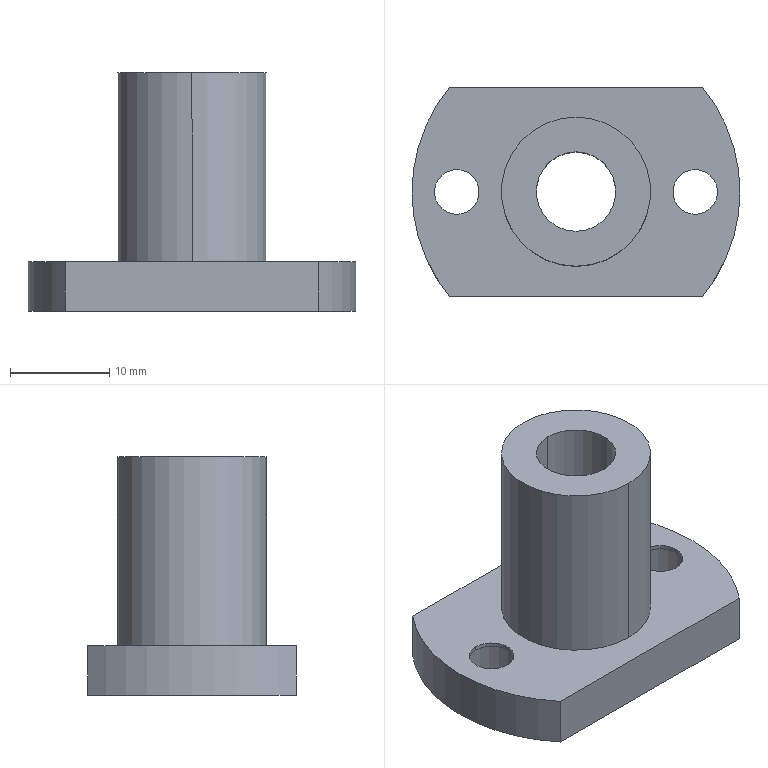Component | SolidWorks | LinearBearing8uu-1 | 1 solid | 21 faces | box 33 x 21 x 24 mm | volume 4890 mm3 | cylinder 14 | plane 7 | commonest cylinder face diameters 8 x6 4.5 x4 15 x2 33 x2
build123d program:
from build123d import *

# Parameters (mm, degrees)
SKETCH2_W                                         = 10.005
SKETCH2_H                                         = 30.735
SKETCH2_W_2                                       = 17.846
SKETCH2_H_2                                       = 33.574
CUT_EXTRUDE1_DEPTH                                = 10
HOLE_SIZE_ACCORDING_TO_HEXAGON_SOCKET_D           = 4.5
HOLE_SIZE_ACCORDING_TO_HEXAGON_SOCKET_DEPTH       = 22.25
HOLE_SIZE_ACCORDING_TO_HEXAGON_SOCKET_CBORE_D     = 8
HOLE_SIZE_ACCORDING_TO_HEXAGON_SOCKET_CBORE_DEPTH = 4.6
HOLE_SIZE_ACCORDING_TO_HEXAGON_SOCKET_TIP         = 1.352


with BuildPart() as part:
    # Sketch1 → Revolve1 (revolve)
    with BuildSketch(Plane.XY, mode=Mode.PRIVATE) as revolve1_sk:
        Polygon((0, 4), (0, 16.5), (5, 16.5), (5, 7.5), (24, 7.5), (24, 4), align=None)
    revolve(revolve1_sk.sketch.rotate(Axis((-24.161, 0, 0), (1, 0, 0)), 90), axis=Axis((-24.161, 0, 0), (1, 0, 0)))

    # Sketch2 → Cut-Extrude1 (cut)
    with BuildSketch(Plane.ZY):
        with Locations((-15.502, 0.676)):
            Rectangle(SKETCH2_W, SKETCH2_H)
        with Locations((19.423, 0.9239)):
            Rectangle(SKETCH2_W_2, SKETCH2_H_2)
    extrude(amount=-CUT_EXTRUDE1_DEPTH, mode=Mode.SUBTRACT)

    # Hole Size _According to_ Hexagon Socket
    with Locations(Plane(origin=(0, 12, 0), x_dir=(0, 0, -1), z_dir=(-1, 0, 0))):
        with Locations((0, 0), (0, 24)):
            CounterBoreHole(HOLE_SIZE_ACCORDING_TO_HEXAGON_SOCKET_D / 2, HOLE_SIZE_ACCORDING_TO_HEXAGON_SOCKET_CBORE_D / 2, HOLE_SIZE_ACCORDING_TO_HEXAGON_SOCKET_CBORE_DEPTH, depth=HOLE_SIZE_ACCORDING_TO_HEXAGON_SOCKET_DEPTH)
            with Locations((0, 0, -(HOLE_SIZE_ACCORDING_TO_HEXAGON_SOCKET_DEPTH + HOLE_SIZE_ACCORDING_TO_HEXAGON_SOCKET_TIP / 2))):  # 118° drill point
                Cone(0, HOLE_SIZE_ACCORDING_TO_HEXAGON_SOCKET_D / 2, HOLE_SIZE_ACCORDING_TO_HEXAGON_SOCKET_TIP, mode=Mode.SUBTRACT)


solid = part.part

# Placed as in the assembly
solid = solid.moved(Location((30, -219.228, 51), (90, 0, 90)))
STEP:
#1=COLOUR_RGB('',0.7922,0.8196,0.9333);
#2=FILL_AREA_STYLE_COLOUR('',#1);
#3=FILL_AREA_STYLE('',(#2));
#4=SURFACE_STYLE_FILL_AREA(#3);
#5=SURFACE_SIDE_STYLE('',(#4));
#6=SURFACE_STYLE_USAGE(.BOTH.,#5);
#7=PRESENTATION_STYLE_ASSIGNMENT((#6));
#8=CARTESIAN_POINT('',(0.7087,-8.474,2.189));
#9=VERTEX_POINT('',#8);
#10=CARTESIAN_POINT('',(0.7087,-8.789,2.189));
#11=VERTEX_POINT('',#10);
#12=CARTESIAN_POINT('',(0.7087,-8.631,2.189));
#13=DIRECTION('',(0.,0.,-1.));
#14=DIRECTION('',(0.,-1.,0.));
#15=AXIS2_PLACEMENT_3D('',#12,#13,#14);
#16=CIRCLE('',#15,0.1575);
#17=EDGE_CURVE('',#9,#11,#16,.T.);
#18=ORIENTED_EDGE('',*,*,#17,.F.);
#19=CARTESIAN_POINT('',(0.7087,-8.474,2.008));
#20=VERTEX_POINT('',#19);
#21=CARTESIAN_POINT('',(0.7087,-8.474,2.008));
#22=DIRECTION('',(0.,0.,-1.));
#23=VECTOR('',#22,39.37);
#24=LINE('',#21,#23);
#25=EDGE_CURVE('',#9,#20,#24,.T.);
#26=ORIENTED_EDGE('',*,*,#25,.T.);
#27=CARTESIAN_POINT('',(0.7087,-8.789,2.008));
#28=VERTEX_POINT('',#27);
#29=CARTESIAN_POINT('',(0.7087,-8.631,2.008));
#30=DIRECTION('',(0.,0.,-1.));
#31=DIRECTION('',(0.,-1.,0.));
#32=AXIS2_PLACEMENT_3D('',#29,#30,#31);
#33=CIRCLE('',#32,0.1575);
#34=EDGE_CURVE('',#20,#28,#33,.T.);
#35=ORIENTED_EDGE('',*,*,#34,.T.);
#36=CARTESIAN_POINT('',(0.7087,-8.789,2.008));
#37=DIRECTION('',(0.,0.,-1.));
#38=VECTOR('',#37,39.37);
#39=LINE('',#36,#38);
#40=EDGE_CURVE('',#11,#28,#39,.T.);
#41=ORIENTED_EDGE('',*,*,#40,.F.);
#42=EDGE_LOOP('',(#18,#26,#35,#41));
#43=FACE_OUTER_BOUND('',#42,.T.);
#44=CARTESIAN_POINT('',(0.7087,-8.631,2.008));
#45=DIRECTION('',(0.,0.,-1.));
#46=DIRECTION('',(0.,-1.,0.));
#47=AXIS2_PLACEMENT_3D('',#44,#45,#46);
#48=CYLINDRICAL_SURFACE('',#47,0.1575);
#49=ADVANCED_FACE('',(#43),#48,.F.);
#50=CARTESIAN_POINT('',(0.7087,-8.542,2.205));
#51=VERTEX_POINT('',#50);
#52=CARTESIAN_POINT('',(0.7087,-8.72,2.205));
#53=VERTEX_POINT('',#52);
#54=CARTESIAN_POINT('',(0.7087,-8.631,2.205));
#55=DIRECTION('',(0.,0.,-1.));
#56=DIRECTION('',(0.,-1.,0.));
#57=AXIS2_PLACEMENT_3D('',#54,#55,#56);
#58=CIRCLE('',#57,0.08858);
#59=EDGE_CURVE('',#51,#53,#58,.T.);
#60=ORIENTED_EDGE('',*,*,#59,.F.);
#61=CARTESIAN_POINT('',(0.7087,-8.542,2.189));
#62=VERTEX_POINT('',#61);
#63=CARTESIAN_POINT('',(0.7087,-8.542,2.008));
#64=DIRECTION('',(0.,0.,-1.));
#65=VECTOR('',#64,39.37);
#66=LINE('',#63,#65);
#67=EDGE_CURVE('',#51,#62,#66,.T.);
#68=ORIENTED_EDGE('',*,*,#67,.T.);
#69=CARTESIAN_POINT('',(0.7087,-8.72,2.189));
#70=VERTEX_POINT('',#69);
#71=CARTESIAN_POINT('',(0.7087,-8.631,2.189));
#72=DIRECTION('',(0.,0.,-1.));
#73=DIRECTION('',(0.,-1.,0.));
#74=AXIS2_PLACEMENT_3D('',#71,#72,#73);
#75=CIRCLE('',#74,0.08858);
#76=EDGE_CURVE('',#62,#70,#75,.T.);
#77=ORIENTED_EDGE('',*,*,#76,.T.);
#78=CARTESIAN_POINT('',(0.7087,-8.72,2.008));
#79=DIRECTION('',(0.,0.,-1.));
#80=VECTOR('',#79,39.37);
#81=LINE('',#78,#80);
#82=EDGE_CURVE('',#53,#70,#81,.T.);
#83=ORIENTED_EDGE('',*,*,#82,.F.);
#84=EDGE_LOOP('',(#60,#68,#77,#83));
#85=FACE_OUTER_BOUND('',#84,.T.);
#86=CARTESIAN_POINT('',(0.7087,-8.631,2.008));
#87=DIRECTION('',(0.,0.,-1.));
#88=DIRECTION('',(0.,-1.,0.));
#89=AXIS2_PLACEMENT_3D('',#86,#87,#88);
#90=CYLINDRICAL_SURFACE('',#89,0.08858);
#91=ADVANCED_FACE('',(#85),#90,.F.);
#92=CARTESIAN_POINT('',(1.654,-8.474,2.189));
#93=VERTEX_POINT('',#92);
#94=CARTESIAN_POINT('',(1.654,-8.789,2.189));
#95=VERTEX_POINT('',#94);
#96=CARTESIAN_POINT('',(1.654,-8.631,2.189));
#97=DIRECTION('',(0.,0.,-1.));
#98=DIRECTION('',(0.,-1.,0.));
#99=AXIS2_PLACEMENT_3D('',#96,#97,#98);
#100=CIRCLE('',#99,0.1575);
#101=EDGE_CURVE('',#93,#95,#100,.T.);
#102=ORIENTED_EDGE('',*,*,#101,.F.);
#103=CARTESIAN_POINT('',(1.654,-8.474,2.008));
#104=VERTEX_POINT('',#103);
#105=CARTESIAN_POINT('',(1.654,-8.474,2.008));
#106=DIRECTION('',(0.,0.,-1.));
#107=VECTOR('',#106,39.37);
#108=LINE('',#105,#107);
#109=EDGE_CURVE('',#93,#104,#108,.T.);
#110=ORIENTED_EDGE('',*,*,#109,.T.);
#111=CARTESIAN_POINT('',(1.654,-8.789,2.008));
#112=VERTEX_POINT('',#111);
#113=CARTESIAN_POINT('',(1.654,-8.631,2.008));
#114=DIRECTION('',(0.,0.,-1.));
#115=DIRECTION('',(0.,-1.,0.));
#116=AXIS2_PLACEMENT_3D('',#113,#114,#115);
#117=CIRCLE('',#116,0.1575);
#118=EDGE_CURVE('',#104,#112,#117,.T.);
#119=ORIENTED_EDGE('',*,*,#118,.T.);
#120=CARTESIAN_POINT('',(1.654,-8.789,2.008));
#121=DIRECTION('',(0.,0.,-1.));
#122=VECTOR('',#121,39.37);
#123=LINE('',#120,#122);
#124=EDGE_CURVE('',#95,#112,#123,.T.);
#125=ORIENTED_EDGE('',*,*,#124,.F.);
#126=EDGE_LOOP('',(#102,#110,#119,#125));
#127=FACE_OUTER_BOUND('',#126,.T.);
#128=CARTESIAN_POINT('',(1.654,-8.631,2.008));
#129=DIRECTION('',(0.,0.,-1.));
#130=DIRECTION('',(0.,-1.,0.));
#131=AXIS2_PLACEMENT_3D('',#128,#129,#130);
#132=CYLINDRICAL_SURFACE('',#131,0.1575);
#133=ADVANCED_FACE('',(#127),#132,.F.);
#134=CARTESIAN_POINT('',(1.654,-8.542,2.205));
#135=VERTEX_POINT('',#134);
#136=CARTESIAN_POINT('',(1.654,-8.72,2.205));
#137=VERTEX_POINT('',#136);
#138=CARTESIAN_POINT('',(1.654,-8.631,2.205));
#139=DIRECTION('',(0.,0.,-1.));
#140=DIRECTION('',(0.,-1.,0.));
#141=AXIS2_PLACEMENT_3D('',#138,#139,#140);
#142=CIRCLE('',#141,0.08858);
#143=EDGE_CURVE('',#135,#137,#142,.T.);
#144=ORIENTED_EDGE('',*,*,#143,.F.);
#145=CARTESIAN_POINT('',(1.654,-8.542,2.189));
#146=VERTEX_POINT('',#145);
#147=CARTESIAN_POINT('',(1.654,-8.542,2.008));
#148=DIRECTION('',(0.,0.,-1.));
#149=VECTOR('',#148,39.37);
#150=LINE('',#147,#149);
#151=EDGE_CURVE('',#135,#146,#150,.T.);
#152=ORIENTED_EDGE('',*,*,#151,.T.);
#153=CARTESIAN_POINT('',(1.654,-8.72,2.189));
#154=VERTEX_POINT('',#153);
#155=CARTESIAN_POINT('',(1.654,-8.631,2.189));
#156=DIRECTION('',(0.,0.,-1.));
#157=DIRECTION('',(0.,-1.,0.));
#158=AXIS2_PLACEMENT_3D('',#155,#156,#157);
#159=CIRCLE('',#158,0.08858);
#160=EDGE_CURVE('',#146,#154,#159,.T.);
#161=ORIENTED_EDGE('',*,*,#160,.T.);
#162=CARTESIAN_POINT('',(1.654,-8.72,2.008));
#163=DIRECTION('',(0.,0.,-1.));
#164=VECTOR('',#163,39.37);
#165=LINE('',#162,#164);
#166=EDGE_CURVE('',#137,#154,#165,.T.);
#167=ORIENTED_EDGE('',*,*,#166,.F.);
#168=EDGE_LOOP('',(#144,#152,#161,#167));
#169=FACE_OUTER_BOUND('',#168,.T.);
#170=CARTESIAN_POINT('',(1.654,-8.631,2.008));
#171=DIRECTION('',(0.,0.,-1.));
#172=DIRECTION('',(0.,-1.,0.));
#173=AXIS2_PLACEMENT_3D('',#170,#171,#172);
#174=CYLINDRICAL_SURFACE('',#173,0.08858);
#175=ADVANCED_FACE('',(#169),#174,.F.);
#176=CARTESIAN_POINT('',(1.181,-8.926,2.953));
#177=VERTEX_POINT('',#176);
#178=CARTESIAN_POINT('',(1.181,-8.336,2.953));
#179=VERTEX_POINT('',#178);
#180=CARTESIAN_POINT('',(1.181,-8.631,2.953));
#181=DIRECTION('',(0.,0.,-1.));
#182=DIRECTION('',(-0.,-1.,0.));
#183=AXIS2_PLACEMENT_3D('',#180,#181,#182);
#184=CIRCLE('',#183,0.2953);
#185=EDGE_CURVE('',#177,#179,#184,.T.);
#186=ORIENTED_EDGE('',*,*,#185,.T.);
#187=CARTESIAN_POINT('',(1.181,-8.336,2.205));
#188=VERTEX_POINT('',#187);
#189=CARTESIAN_POINT('',(1.181,-8.336,1.057));
#190=DIRECTION('',(0.,0.,-1.));
#191=VECTOR('',#190,39.37);
#192=LINE('',#189,#191);
#193=EDGE_CURVE('',#179,#188,#192,.T.);
#194=ORIENTED_EDGE('',*,*,#193,.T.);
#195=CARTESIAN_POINT('',(1.181,-8.926,2.205));
#196=VERTEX_POINT('',#195);
#197=CARTESIAN_POINT('',(1.181,-8.631,2.205));
#198=DIRECTION('',(0.,0.,-1.));
#199=DIRECTION('',(-0.,-1.,0.));
#200=AXIS2_PLACEMENT_3D('',#197,#198,#199);
#201=CIRCLE('',#200,0.2953);
#202=EDGE_CURVE('',#196,#188,#201,.T.);
#203=ORIENTED_EDGE('',*,*,#202,.F.);
#204=CARTESIAN_POINT('',(1.181,-8.926,1.057));
#205=DIRECTION('',(0.,0.,-1.));
#206=VECTOR('',#205,39.37);
#207=LINE('',#204,#206);
#208=EDGE_CURVE('',#177,#196,#207,.T.);
#209=ORIENTED_EDGE('',*,*,#208,.F.);
#210=EDGE_LOOP('',(#186,#194,#203,#209));
#211=FACE_OUTER_BOUND('',#210,.T.);
#212=CARTESIAN_POINT('',(1.181,-8.631,1.057));
#213=DIRECTION('',(0.,0.,-1.));
#214=DIRECTION('',(-0.,-1.,-0.));
#215=AXIS2_PLACEMENT_3D('',#212,#213,#214);
#216=CYLINDRICAL_SURFACE('',#215,0.2953);
#217=ADVANCED_FACE('',(#211),#216,.T.);
#218=CARTESIAN_POINT('',(1.181,-8.474,2.953));
#219=VERTEX_POINT('',#218);
#220=CARTESIAN_POINT('',(1.181,-8.789,2.953));
#221=VERTEX_POINT('',#220);
#222=CARTESIAN_POINT('',(1.181,-8.631,2.953));
#223=DIRECTION('',(0.,0.,-1.));
#224=DIRECTION('',(0.,-1.,0.));
#225=AXIS2_PLACEMENT_3D('',#222,#223,#224);
#226=CIRCLE('',#225,0.1575);
#227=EDGE_CURVE('',#219,#221,#226,.T.);
#228=ORIENTED_EDGE('',*,*,#227,.F.);
#229=CARTESIAN_POINT('',(1.181,-8.474,2.008));
#230=VERTEX_POINT('',#229);
#231=CARTESIAN_POINT('',(1.181,-8.474,1.057));
#232=DIRECTION('',(0.,0.,-1.));
#233=VECTOR('',#232,39.37);
#234=LINE('',#231,#233);
#235=EDGE_CURVE('',#219,#230,#234,.T.);
#236=ORIENTED_EDGE('',*,*,#235,.T.);
#237=CARTESIAN_POINT('',(1.181,-8.789,2.008));
#238=VERTEX_POINT('',#237);
#239=CARTESIAN_POINT('',(1.181,-8.631,2.008));
#240=DIRECTION('',(0.,0.,-1.));
#241=DIRECTION('',(0.,-1.,0.));
#242=AXIS2_PLACEMENT_3D('',#239,#240,#241);
#243=CIRCLE('',#242,0.1575);
#244=EDGE_CURVE('',#230,#238,#243,.T.);
#245=ORIENTED_EDGE('',*,*,#244,.T.);
#246=CARTESIAN_POINT('',(1.181,-8.789,1.057));
#247=DIRECTION('',(0.,0.,-1.));
#248=VECTOR('',#247,39.37);
#249=LINE('',#246,#248);
#250=EDGE_CURVE('',#221,#238,#249,.T.);
#251=ORIENTED_EDGE('',*,*,#250,.F.);
#252=EDGE_LOOP('',(#228,#236,#245,#251));
#253=FACE_OUTER_BOUND('',#252,.T.);
#254=CARTESIAN_POINT('',(1.181,-8.631,1.057));
#255=DIRECTION('',(0.,0.,-1.));
#256=DIRECTION('',(0.,-1.,0.));
#257=AXIS2_PLACEMENT_3D('',#254,#255,#256);
#258=CYLINDRICAL_SURFACE('',#257,0.1575);
#259=ADVANCED_FACE('',(#253),#258,.F.);
#260=CARTESIAN_POINT('',(1.682,-8.218,2.205));
#261=VERTEX_POINT('',#260);
#262=CARTESIAN_POINT('',(1.682,-9.044,2.205));
#263=VERTEX_POINT('',#262);
#264=CARTESIAN_POINT('',(1.181,-8.631,2.205));
#265=DIRECTION('',(0.,0.,-1.));
#266=DIRECTION('',(-0.,-1.,-0.));
#267=AXIS2_PLACEMENT_3D('',#264,#265,#266);
#268=CIRCLE('',#267,0.6496);
#269=EDGE_CURVE('',#261,#263,#268,.T.);
#270=ORIENTED_EDGE('',*,*,#269,.T.);
#271=CARTESIAN_POINT('',(1.682,-9.044,2.008));
#272=VERTEX_POINT('',#271);
#273=CARTESIAN_POINT('',(1.682,-9.044,1.057));
#274=DIRECTION('',(0.,0.,-1.));
#275=VECTOR('',#274,39.37);
#276=LINE('',#273,#275);
#277=EDGE_CURVE('',#263,#272,#276,.T.);
#278=ORIENTED_EDGE('',*,*,#277,.T.);
#279=CARTESIAN_POINT('',(1.682,-8.218,2.008));
#280=VERTEX_POINT('',#279);
#281=CARTESIAN_POINT('',(1.181,-8.631,2.008));
#282=DIRECTION('',(0.,0.,-1.));
#283=DIRECTION('',(-0.,-1.,-0.));
#284=AXIS2_PLACEMENT_3D('',#281,#282,#283);
#285=CIRCLE('',#284,0.6496);
#286=EDGE_CURVE('',#280,#272,#285,.T.);
#287=ORIENTED_EDGE('',*,*,#286,.F.);
#288=CARTESIAN_POINT('',(1.682,-8.218,1.057));
#289=DIRECTION('',(-0.,-0.,1.));
#290=VECTOR('',#289,39.37);
#291=LINE('',#288,#290);
#292=EDGE_CURVE('',#280,#261,#291,.T.);
#293=ORIENTED_EDGE('',*,*,#292,.T.);
#294=EDGE_LOOP('',(#270,#278,#287,#293));
#295=FACE_OUTER_BOUND('',#294,.T.);
#296=CARTESIAN_POINT('',(1.181,-8.631,1.057));
#297=DIRECTION('',(0.,0.,-1.));
#298=DIRECTION('',(-0.,-1.,-0.));
#299=AXIS2_PLACEMENT_3D('',#296,#297,#298);
#300=CYLINDRICAL_SURFACE('',#299,0.6496);
#301=ADVANCED_FACE('',(#295),#300,.T.);
#302=ORIENTED_EDGE('',*,*,#235,.F.);
#303=CARTESIAN_POINT('',(1.181,-8.631,2.953));
#304=DIRECTION('',(0.,0.,-1.));
#305=DIRECTION('',(0.,-1.,0.));
#306=AXIS2_PLACEMENT_3D('',#303,#304,#305);
#307=CIRCLE('',#306,0.1575);
#308=EDGE_CURVE('',#221,#219,#307,.T.);
#309=ORIENTED_EDGE('',*,*,#308,.F.);
#310=ORIENTED_EDGE('',*,*,#250,.T.);
#311=CARTESIAN_POINT('',(1.181,-8.631,2.008));
#312=DIRECTION('',(0.,0.,-1.));
#313=DIRECTION('',(0.,-1.,0.));
#314=AXIS2_PLACEMENT_3D('',#311,#312,#313);
#315=CIRCLE('',#314,0.1575);
#316=EDGE_CURVE('',#238,#230,#315,.T.);
#317=ORIENTED_EDGE('',*,*,#316,.T.);
#318=EDGE_LOOP('',(#302,#309,#310,#317));
#319=FACE_OUTER_BOUND('',#318,.T.);
#320=CARTESIAN_POINT('',(1.181,-8.631,1.057));
#321=DIRECTION('',(0.,0.,-1.));
#322=DIRECTION('',(0.,-1.,0.));
#323=AXIS2_PLACEMENT_3D('',#320,#321,#322);
#324=CYLINDRICAL_SURFACE('',#323,0.1575);
#325=ADVANCED_FACE('',(#319),#324,.F.);
#326=CARTESIAN_POINT('',(0.7087,-8.631,2.008));
#327=DIRECTION('',(0.,0.,-1.));
#328=DIRECTION('',(0.,-1.,0.));
#329=AXIS2_PLACEMENT_3D('',#326,#327,#328);
#330=CIRCLE('',#329,0.1575);
#331=EDGE_CURVE('',#28,#20,#330,.T.);
#332=ORIENTED_EDGE('',*,*,#331,.F.);
#333=ORIENTED_EDGE('',*,*,#34,.F.);
#334=EDGE_LOOP('',(#332,#333));
#335=FACE_BOUND('',#334,.T.);
#336=CARTESIAN_POINT('',(1.654,-8.631,2.008));
#337=DIRECTION('',(0.,0.,-1.));
#338=DIRECTION('',(0.,-1.,0.));
#339=AXIS2_PLACEMENT_3D('',#336,#337,#338);
#340=CIRCLE('',#339,0.1575);
#341=EDGE_CURVE('',#112,#104,#340,.T.);
#342=ORIENTED_EDGE('',*,*,#341,.F.);
#343=ORIENTED_EDGE('',*,*,#118,.F.);
#344=EDGE_LOOP('',(#342,#343));
#345=FACE_BOUND('',#344,.T.);
#346=ORIENTED_EDGE('',*,*,#316,.F.);
#347=ORIENTED_EDGE('',*,*,#244,.F.);
#348=EDGE_LOOP('',(#346,#347));
#349=FACE_BOUND('',#348,.T.);
#350=ORIENTED_EDGE('',*,*,#286,.T.);
#351=CARTESIAN_POINT('',(0.68,-9.044,2.008));
#352=VERTEX_POINT('',#351);
#353=CARTESIAN_POINT('',(0.4838,-9.044,2.008));
#354=DIRECTION('',(1.,-0.,0.));
#355=VECTOR('',#354,39.37);
#356=LINE('',#353,#355);
#357=EDGE_CURVE('',#352,#272,#356,.T.);
#358=ORIENTED_EDGE('',*,*,#357,.F.);
#359=CARTESIAN_POINT('',(0.68,-8.218,2.008));
#360=VERTEX_POINT('',#359);
#361=CARTESIAN_POINT('',(1.181,-8.631,2.008));
#362=DIRECTION('',(0.,0.,-1.));
#363=DIRECTION('',(-0.,-1.,-0.));
#364=AXIS2_PLACEMENT_3D('',#361,#362,#363);
#365=CIRCLE('',#364,0.6496);
#366=EDGE_CURVE('',#352,#360,#365,.T.);
#367=ORIENTED_EDGE('',*,*,#366,.T.);
#368=CARTESIAN_POINT('',(0.5495,-8.218,2.008));
#369=DIRECTION('',(-1.,0.,-0.));
#370=VECTOR('',#369,39.37);
#371=LINE('',#368,#370);
#372=EDGE_CURVE('',#280,#360,#371,.T.);
#373=ORIENTED_EDGE('',*,*,#372,.F.);
#374=EDGE_LOOP('',(#350,#358,#367,#373));
#375=FACE_OUTER_BOUND('',#374,.T.);
#376=CARTESIAN_POINT('',(1.024,-8.631,2.008));
#377=DIRECTION('',(-0.,-0.,1.));
#378=DIRECTION('',(0.,1.,0.));
#379=AXIS2_PLACEMENT_3D('',#376,#377,#378);
#380=PLANE('',#379);
#381=ADVANCED_FACE('',(#335,#345,#349,#375),#380,.F.);
#382=ORIENTED_EDGE('',*,*,#366,.F.);
#383=CARTESIAN_POINT('',(0.68,-9.044,2.205));
#384=VERTEX_POINT('',#383);
#385=CARTESIAN_POINT('',(0.68,-9.044,1.057));
#386=DIRECTION('',(-0.,-0.,1.));
#387=VECTOR('',#386,39.37);
#388=LINE('',#385,#387);
#389=EDGE_CURVE('',#352,#384,#388,.T.);
#390=ORIENTED_EDGE('',*,*,#389,.T.);
#391=CARTESIAN_POINT('',(0.68,-8.218,2.205));
#392=VERTEX_POINT('',#391);
#393=CARTESIAN_POINT('',(1.181,-8.631,2.205));
#394=DIRECTION('',(0.,0.,-1.));
#395=DIRECTION('',(-0.,-1.,-0.));
#396=AXIS2_PLACEMENT_3D('',#393,#394,#395);
#397=CIRCLE('',#396,0.6496);
#398=EDGE_CURVE('',#384,#392,#397,.T.);
#399=ORIENTED_EDGE('',*,*,#398,.T.);
#400=CARTESIAN_POINT('',(0.68,-8.218,1.057));
#401=DIRECTION('',(0.,0.,-1.));
#402=VECTOR('',#401,39.37);
#403=LINE('',#400,#402);
#404=EDGE_CURVE('',#392,#360,#403,.T.);
#405=ORIENTED_EDGE('',*,*,#404,.T.);
#406=EDGE_LOOP('',(#382,#390,#399,#405));
#407=FACE_OUTER_BOUND('',#406,.T.);
#408=CARTESIAN_POINT('',(1.181,-8.631,1.057));
#409=DIRECTION('',(0.,0.,-1.));
#410=DIRECTION('',(-0.,-1.,-0.));
#411=AXIS2_PLACEMENT_3D('',#408,#409,#410);
#412=CYLINDRICAL_SURFACE('',#411,0.6496);
#413=ADVANCED_FACE('',(#407),#412,.T.);
#414=CARTESIAN_POINT('',(0.7087,-8.631,2.205));
#415=DIRECTION('',(0.,0.,-1.));
#416=DIRECTION('',(0.,-1.,0.));
#417=AXIS2_PLACEMENT_3D('',#414,#415,#416);
#418=CIRCLE('',#417,0.08858);
#419=EDGE_CURVE('',#53,#51,#418,.T.);
#420=ORIENTED_EDGE('',*,*,#419,.T.);
#421=ORIENTED_EDGE('',*,*,#59,.T.);
#422=EDGE_LOOP('',(#420,#421));
#423=FACE_BOUND('',#422,.T.);
#424=CARTESIAN_POINT('',(1.654,-8.631,2.205));
#425=DIRECTION('',(0.,0.,-1.));
#426=DIRECTION('',(0.,-1.,0.));
#427=AXIS2_PLACEMENT_3D('',#424,#425,#426);
#428=CIRCLE('',#427,0.08858);
#429=EDGE_CURVE('',#137,#135,#428,.T.);
#430=ORIENTED_EDGE('',*,*,#429,.T.);
#431=ORIENTED_EDGE('',*,*,#143,.T.);
#432=EDGE_LOOP('',(#430,#431));
#433=FACE_BOUND('',#432,.T.);
#434=ORIENTED_EDGE('',*,*,#398,.F.);
#435=CARTESIAN_POINT('',(0.5315,-9.044,2.205));
#436=DIRECTION('',(1.,-0.,0.));
#437=VECTOR('',#436,39.37);
#438=LINE('',#435,#437);
#439=EDGE_CURVE('',#384,#263,#438,.T.);
#440=ORIENTED_EDGE('',*,*,#439,.T.);
#441=ORIENTED_EDGE('',*,*,#269,.F.);
#442=CARTESIAN_POINT('',(0.5315,-8.218,2.205));
#443=DIRECTION('',(-1.,0.,-0.));
#444=VECTOR('',#443,39.37);
#445=LINE('',#442,#444);
#446=EDGE_CURVE('',#261,#392,#445,.T.);
#447=ORIENTED_EDGE('',*,*,#446,.T.);
#448=EDGE_LOOP('',(#434,#440,#441,#447));
#449=FACE_OUTER_BOUND('',#448,.T.);
#450=ORIENTED_EDGE('',*,*,#202,.T.);
#451=CARTESIAN_POINT('',(1.181,-8.631,2.205));
#452=DIRECTION('',(0.,0.,-1.));
#453=DIRECTION('',(-0.,-1.,0.));
#454=AXIS2_PLACEMENT_3D('',#451,#452,#453);
#455=CIRCLE('',#454,0.2953);
#456=EDGE_CURVE('',#188,#196,#455,.T.);
#457=ORIENTED_EDGE('',*,*,#456,.T.);
#458=EDGE_LOOP('',(#450,#457));
#459=FACE_BOUND('',#458,.T.);
#460=CARTESIAN_POINT('',(0.5315,-8.631,2.205));
#461=DIRECTION('',(0.,0.,-1.));
#462=DIRECTION('',(-0.,-1.,-0.));
#463=AXIS2_PLACEMENT_3D('',#460,#461,#462);
#464=PLANE('',#463);
#465=ADVANCED_FACE('',(#423,#433,#449,#459),#464,.F.);
#466=ORIENTED_EDGE('',*,*,#193,.F.);
#467=CARTESIAN_POINT('',(1.181,-8.631,2.953));
#468=DIRECTION('',(0.,0.,-1.));
#469=DIRECTION('',(-0.,-1.,0.));
#470=AXIS2_PLACEMENT_3D('',#467,#468,#469);
#471=CIRCLE('',#470,0.2953);
#472=EDGE_CURVE('',#179,#177,#471,.T.);
#473=ORIENTED_EDGE('',*,*,#472,.T.);
#474=ORIENTED_EDGE('',*,*,#208,.T.);
#475=ORIENTED_EDGE('',*,*,#456,.F.);
#476=EDGE_LOOP('',(#466,#473,#474,#475));
#477=FACE_OUTER_BOUND('',#476,.T.);
#478=CARTESIAN_POINT('',(1.181,-8.631,1.057));
#479=DIRECTION('',(0.,0.,-1.));
#480=DIRECTION('',(-0.,-1.,-0.));
#481=AXIS2_PLACEMENT_3D('',#478,#479,#480);
#482=CYLINDRICAL_SURFACE('',#481,0.2953);
#483=ADVANCED_FACE('',(#477),#482,.T.);
#484=ORIENTED_EDGE('',*,*,#185,.F.);
#485=ORIENTED_EDGE('',*,*,#472,.F.);
#486=EDGE_LOOP('',(#484,#485));
#487=FACE_OUTER_BOUND('',#486,.T.);
#488=ORIENTED_EDGE('',*,*,#308,.T.);
#489=ORIENTED_EDGE('',*,*,#227,.T.);
#490=EDGE_LOOP('',(#488,#489));
#491=FACE_BOUND('',#490,.T.);
#492=CARTESIAN_POINT('',(0.8858,-8.631,2.953));
#493=DIRECTION('',(0.,0.,-1.));
#494=DIRECTION('',(-0.,-1.,-0.));
#495=AXIS2_PLACEMENT_3D('',#492,#493,#494);
#496=PLANE('',#495);
#497=ADVANCED_FACE('',(#487,#491),#496,.F.);
#498=ORIENTED_EDGE('',*,*,#446,.F.);
#499=ORIENTED_EDGE('',*,*,#292,.F.);
#500=ORIENTED_EDGE('',*,*,#372,.T.);
#501=ORIENTED_EDGE('',*,*,#404,.F.);
#502=EDGE_LOOP('',(#498,#499,#500,#501));
#503=FACE_OUTER_BOUND('',#502,.T.);
#504=CARTESIAN_POINT('',(0.5495,-8.218,2.402));
#505=DIRECTION('',(-0.,-1.,-0.));
#506=DIRECTION('',(1.,-0.,0.));
#507=AXIS2_PLACEMENT_3D('',#504,#505,#506);
#508=PLANE('',#507);
#509=ADVANCED_FACE('',(#503),#508,.F.);
#510=ORIENTED_EDGE('',*,*,#439,.F.);
#511=ORIENTED_EDGE('',*,*,#389,.F.);
#512=ORIENTED_EDGE('',*,*,#357,.T.);
#513=ORIENTED_EDGE('',*,*,#277,.F.);
#514=EDGE_LOOP('',(#510,#511,#512,#513));
#515=FACE_OUTER_BOUND('',#514,.T.);
#516=CARTESIAN_POINT('',(0.4838,-9.044,2.402));
#517=DIRECTION('',(0.,1.,0.));
#518=DIRECTION('',(-1.,0.,-0.));
#519=AXIS2_PLACEMENT_3D('',#516,#517,#518);
#520=PLANE('',#519);
#521=ADVANCED_FACE('',(#515),#520,.F.);
#522=ORIENTED_EDGE('',*,*,#151,.F.);
#523=ORIENTED_EDGE('',*,*,#429,.F.);
#524=ORIENTED_EDGE('',*,*,#166,.T.);
#525=CARTESIAN_POINT('',(1.654,-8.631,2.189));
#526=DIRECTION('',(0.,0.,-1.));
#527=DIRECTION('',(0.,-1.,0.));
#528=AXIS2_PLACEMENT_3D('',#525,#526,#527);
#529=CIRCLE('',#528,0.08858);
#530=EDGE_CURVE('',#154,#146,#529,.T.);
#531=ORIENTED_EDGE('',*,*,#530,.T.);
#532=EDGE_LOOP('',(#522,#523,#524,#531));
#533=FACE_OUTER_BOUND('',#532,.T.);
#534=CARTESIAN_POINT('',(1.654,-8.631,2.008));
#535=DIRECTION('',(0.,0.,-1.));
#536=DIRECTION('',(0.,-1.,0.));
#537=AXIS2_PLACEMENT_3D('',#534,#535,#536);
#538=CYLINDRICAL_SURFACE('',#537,0.08858);
#539=ADVANCED_FACE('',(#533),#538,.F.);
#540=ORIENTED_EDGE('',*,*,#530,.F.);
#541=ORIENTED_EDGE('',*,*,#160,.F.);
#542=EDGE_LOOP('',(#540,#541));
#543=FACE_BOUND('',#542,.T.);
#544=CARTESIAN_POINT('',(1.654,-8.631,2.189));
#545=DIRECTION('',(0.,0.,-1.));
#546=DIRECTION('',(0.,-1.,0.));
#547=AXIS2_PLACEMENT_3D('',#544,#545,#546);
#548=CIRCLE('',#547,0.1575);
#549=EDGE_CURVE('',#95,#93,#548,.T.);
#550=ORIENTED_EDGE('',*,*,#549,.T.);
#551=ORIENTED_EDGE('',*,*,#101,.T.);
#552=EDGE_LOOP('',(#550,#551));
#553=FACE_OUTER_BOUND('',#552,.T.);
#554=CARTESIAN_POINT('',(1.565,-8.631,2.189));
#555=DIRECTION('',(-0.,-0.,1.));
#556=DIRECTION('',(0.,1.,0.));
#557=AXIS2_PLACEMENT_3D('',#554,#555,#556);
#558=PLANE('',#557);
#559=ADVANCED_FACE('',(#543,#553),#558,.F.);
#560=ORIENTED_EDGE('',*,*,#109,.F.);
#561=ORIENTED_EDGE('',*,*,#549,.F.);
#562=ORIENTED_EDGE('',*,*,#124,.T.);
#563=ORIENTED_EDGE('',*,*,#341,.T.);
#564=EDGE_LOOP('',(#560,#561,#562,#563));
#565=FACE_OUTER_BOUND('',#564,.T.);
#566=CARTESIAN_POINT('',(1.654,-8.631,2.008));
#567=DIRECTION('',(0.,0.,-1.));
#568=DIRECTION('',(0.,-1.,0.));
#569=AXIS2_PLACEMENT_3D('',#566,#567,#568);
#570=CYLINDRICAL_SURFACE('',#569,0.1575);
#571=ADVANCED_FACE('',(#565),#570,.F.);
#572=ORIENTED_EDGE('',*,*,#67,.F.);
#573=ORIENTED_EDGE('',*,*,#419,.F.);
#574=ORIENTED_EDGE('',*,*,#82,.T.);
#575=CARTESIAN_POINT('',(0.7087,-8.631,2.189));
#576=DIRECTION('',(0.,0.,-1.));
#577=DIRECTION('',(0.,-1.,0.));
#578=AXIS2_PLACEMENT_3D('',#575,#576,#577);
#579=CIRCLE('',#578,0.08858);
#580=EDGE_CURVE('',#70,#62,#579,.T.);
#581=ORIENTED_EDGE('',*,*,#580,.T.);
#582=EDGE_LOOP('',(#572,#573,#574,#581));
#583=FACE_OUTER_BOUND('',#582,.T.);
#584=CARTESIAN_POINT('',(0.7087,-8.631,2.008));
#585=DIRECTION('',(0.,0.,-1.));
#586=DIRECTION('',(0.,-1.,0.));
#587=AXIS2_PLACEMENT_3D('',#584,#585,#586);
#588=CYLINDRICAL_SURFACE('',#587,0.08858);
#589=ADVANCED_FACE('',(#583),#588,.F.);
#590=ORIENTED_EDGE('',*,*,#580,.F.);
#591=ORIENTED_EDGE('',*,*,#76,.F.);
#592=EDGE_LOOP('',(#590,#591));
#593=FACE_BOUND('',#592,.T.);
#594=CARTESIAN_POINT('',(0.7087,-8.631,2.189));
#595=DIRECTION('',(0.,0.,-1.));
#596=DIRECTION('',(0.,-1.,0.));
#597=AXIS2_PLACEMENT_3D('',#594,#595,#596);
#598=CIRCLE('',#597,0.1575);
#599=EDGE_CURVE('',#11,#9,#598,.T.);
#600=ORIENTED_EDGE('',*,*,#599,.T.);
#601=ORIENTED_EDGE('',*,*,#17,.T.);
#602=EDGE_LOOP('',(#600,#601));
#603=FACE_OUTER_BOUND('',#602,.T.);
#604=CARTESIAN_POINT('',(0.6201,-8.631,2.189));
#605=DIRECTION('',(-0.,-0.,1.));
#606=DIRECTION('',(0.,1.,0.));
#607=AXIS2_PLACEMENT_3D('',#604,#605,#606);
#608=PLANE('',#607);
#609=ADVANCED_FACE('',(#593,#603),#608,.F.);
#610=ORIENTED_EDGE('',*,*,#25,.F.);
#611=ORIENTED_EDGE('',*,*,#599,.F.);
#612=ORIENTED_EDGE('',*,*,#40,.T.);
#613=ORIENTED_EDGE('',*,*,#331,.T.);
#614=EDGE_LOOP('',(#610,#611,#612,#613));
#615=FACE_OUTER_BOUND('',#614,.T.);
#616=CARTESIAN_POINT('',(0.7087,-8.631,2.008));
#617=DIRECTION('',(0.,0.,-1.));
#618=DIRECTION('',(0.,-1.,0.));
#619=AXIS2_PLACEMENT_3D('',#616,#617,#618);
#620=CYLINDRICAL_SURFACE('',#619,0.1575);
#621=ADVANCED_FACE('',(#615),#620,.F.);
#622=CLOSED_SHELL('',(#49,#91,#133,#175,#217,#259,#301,#325,#381,#413,#465,#483,#497,#509,#521,#539,#559,#571,#589,#609,#621));
#623=MANIFOLD_SOLID_BREP('',#622);
#624=STYLED_ITEM('',(#7),#623);
#625=PRESENTATION_LAYER_ASSIGNMENT('','',(#624));
#626=(LENGTH_UNIT()NAMED_UNIT(*)SI_UNIT($,.METRE.));
#627=LENGTH_MEASURE_WITH_UNIT(LENGTH_MEASURE(0.0254),#626);
#628=DIMENSIONAL_EXPONENTS(1.,0.,0.,0.,0.,0.,0.);
#629=(CONVERSION_BASED_UNIT('',#627)LENGTH_UNIT()NAMED_UNIT(#628));
#630=UNCERTAINTY_MEASURE_WITH_UNIT(LENGTH_MEASURE(0.00001),#629,'','');
#631=(NAMED_UNIT(*)PLANE_ANGLE_UNIT()SI_UNIT($,.RADIAN.));
#632=(NAMED_UNIT(*)SI_UNIT($,.STERADIAN.)SOLID_ANGLE_UNIT());
#633=(GEOMETRIC_REPRESENTATION_CONTEXT(3)GLOBAL_UNCERTAINTY_ASSIGNED_CONTEXT((#630))GLOBAL_UNIT_ASSIGNED_CONTEXT((#629,#631,#632))REPRESENTATION_CONTEXT('',''));
#634=MECHANICAL_DESIGN_GEOMETRIC_PRESENTATION_REPRESENTATION('',(#624),#633);
#635=CARTESIAN_POINT('',(0.,0.,0.));
#636=DIRECTION('',(0.,0.,1.));
#637=DIRECTION('',(1.,0.,0.));
#638=AXIS2_PLACEMENT_3D('',#635,#636,#637);
#639=(LENGTH_UNIT()NAMED_UNIT(*)SI_UNIT($,.METRE.));
#640=LENGTH_MEASURE_WITH_UNIT(LENGTH_MEASURE(0.0254),#639);
#641=DIMENSIONAL_EXPONENTS(1.,0.,0.,0.,0.,0.,0.);
#642=(CONVERSION_BASED_UNIT('',#640)LENGTH_UNIT()NAMED_UNIT(#641));
#643=UNCERTAINTY_MEASURE_WITH_UNIT(LENGTH_MEASURE(0.00001),#642,'','');
#644=(NAMED_UNIT(*)PLANE_ANGLE_UNIT()SI_UNIT($,.RADIAN.));
#645=(NAMED_UNIT(*)SI_UNIT($,.STERADIAN.)SOLID_ANGLE_UNIT());
#646=(GEOMETRIC_REPRESENTATION_CONTEXT(3)GLOBAL_UNCERTAINTY_ASSIGNED_CONTEXT((#643))GLOBAL_UNIT_ASSIGNED_CONTEXT((#642,#644,#645))REPRESENTATION_CONTEXT('',''));
#647=ADVANCED_BREP_SHAPE_REPRESENTATION('',(#623,#638),#646);